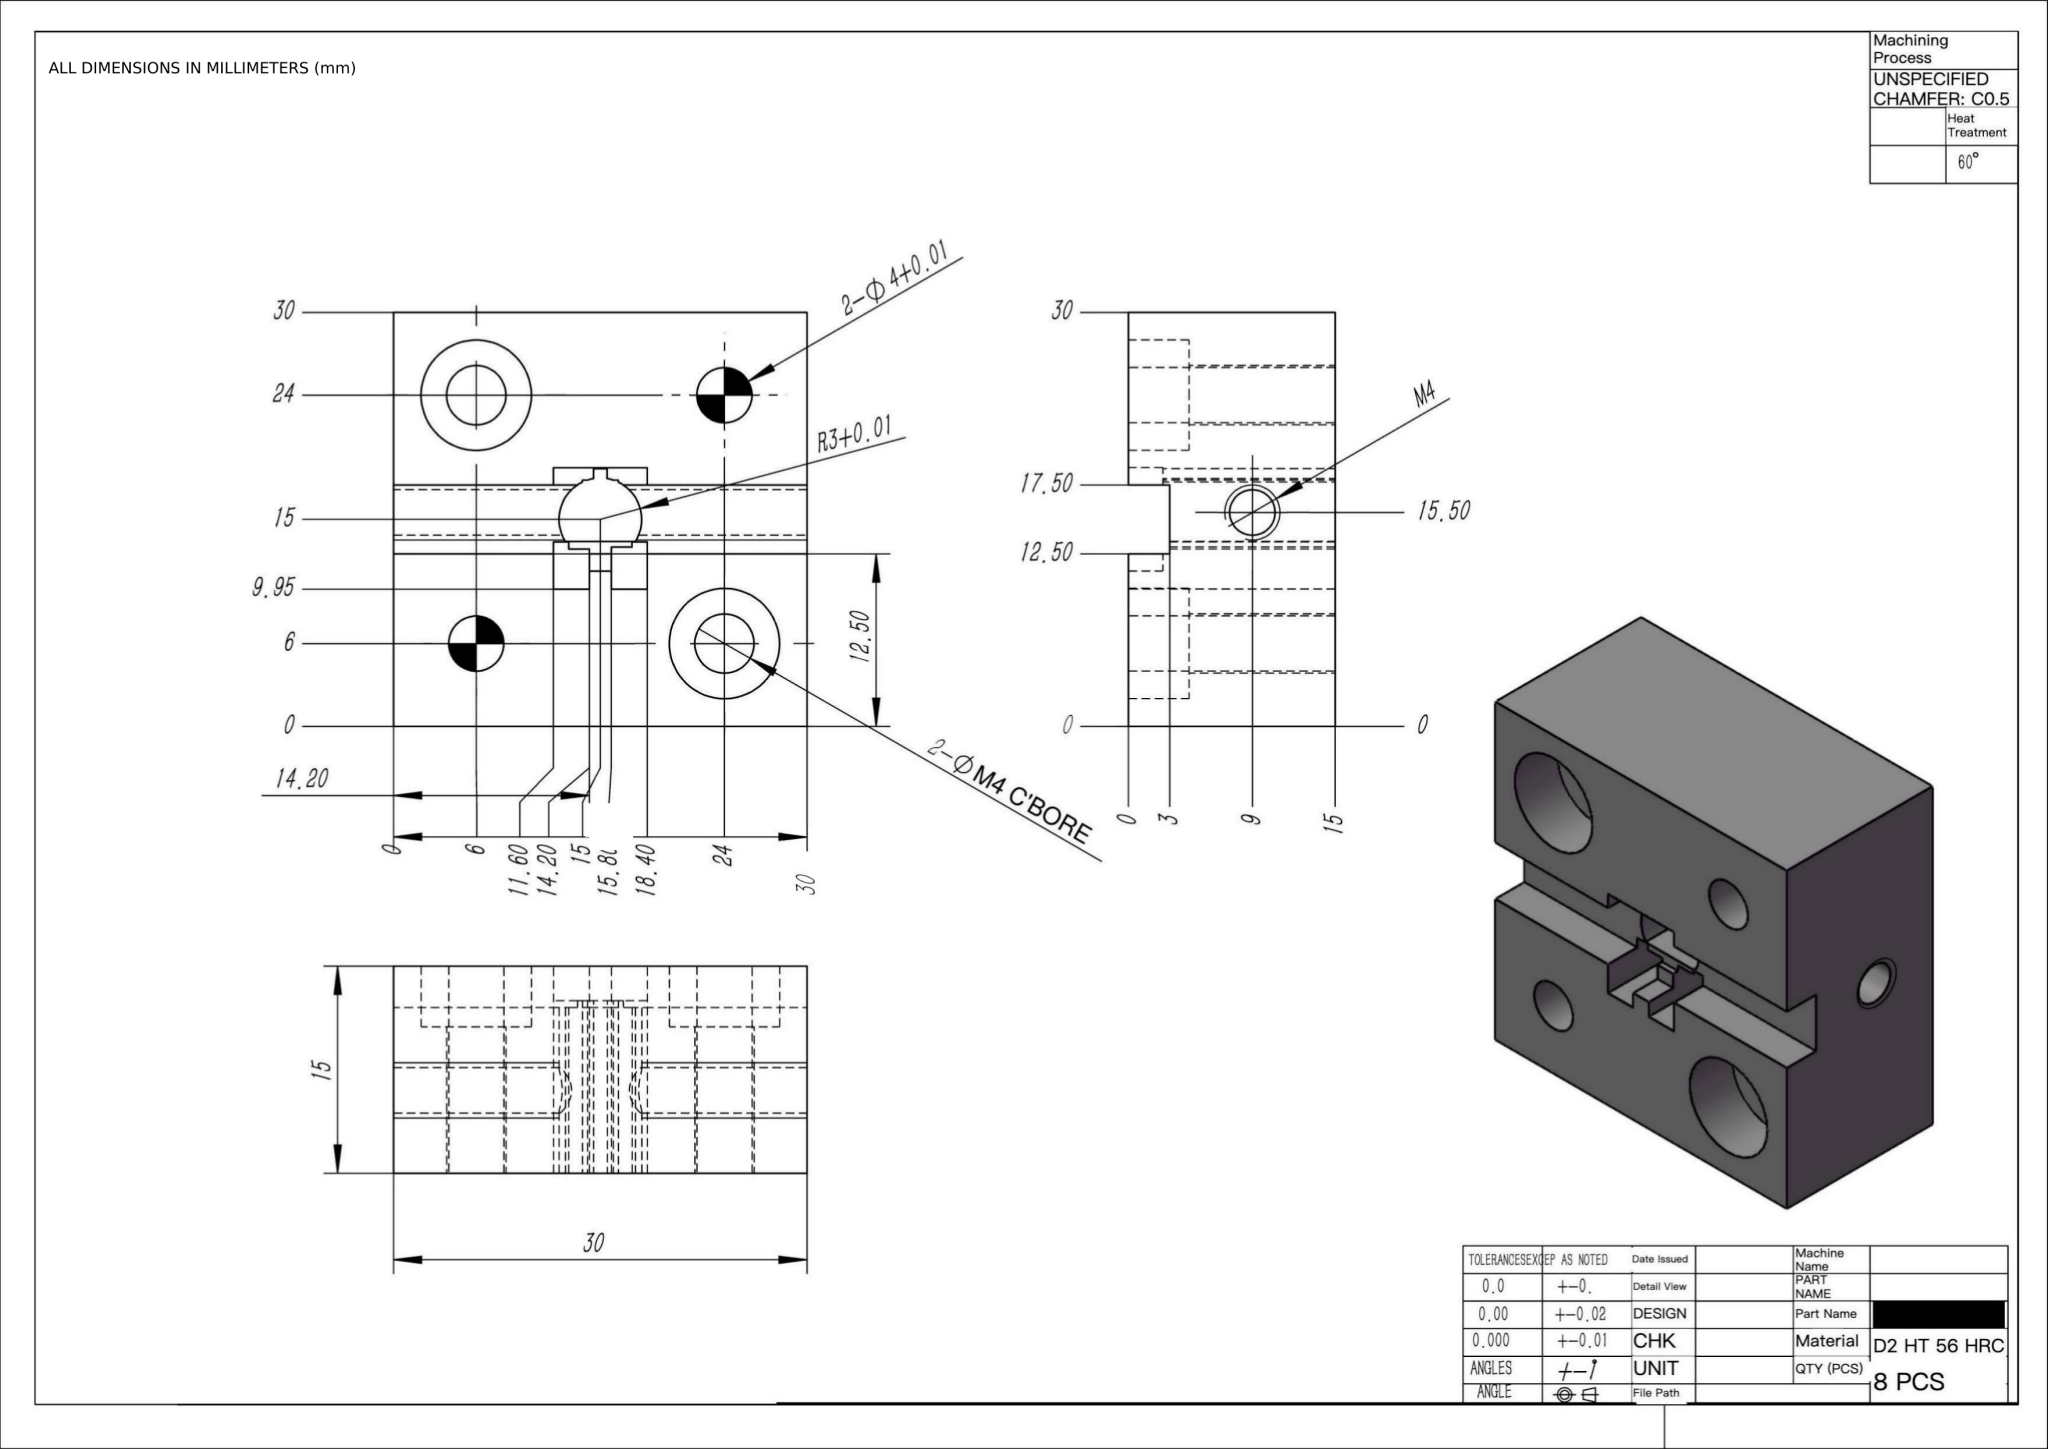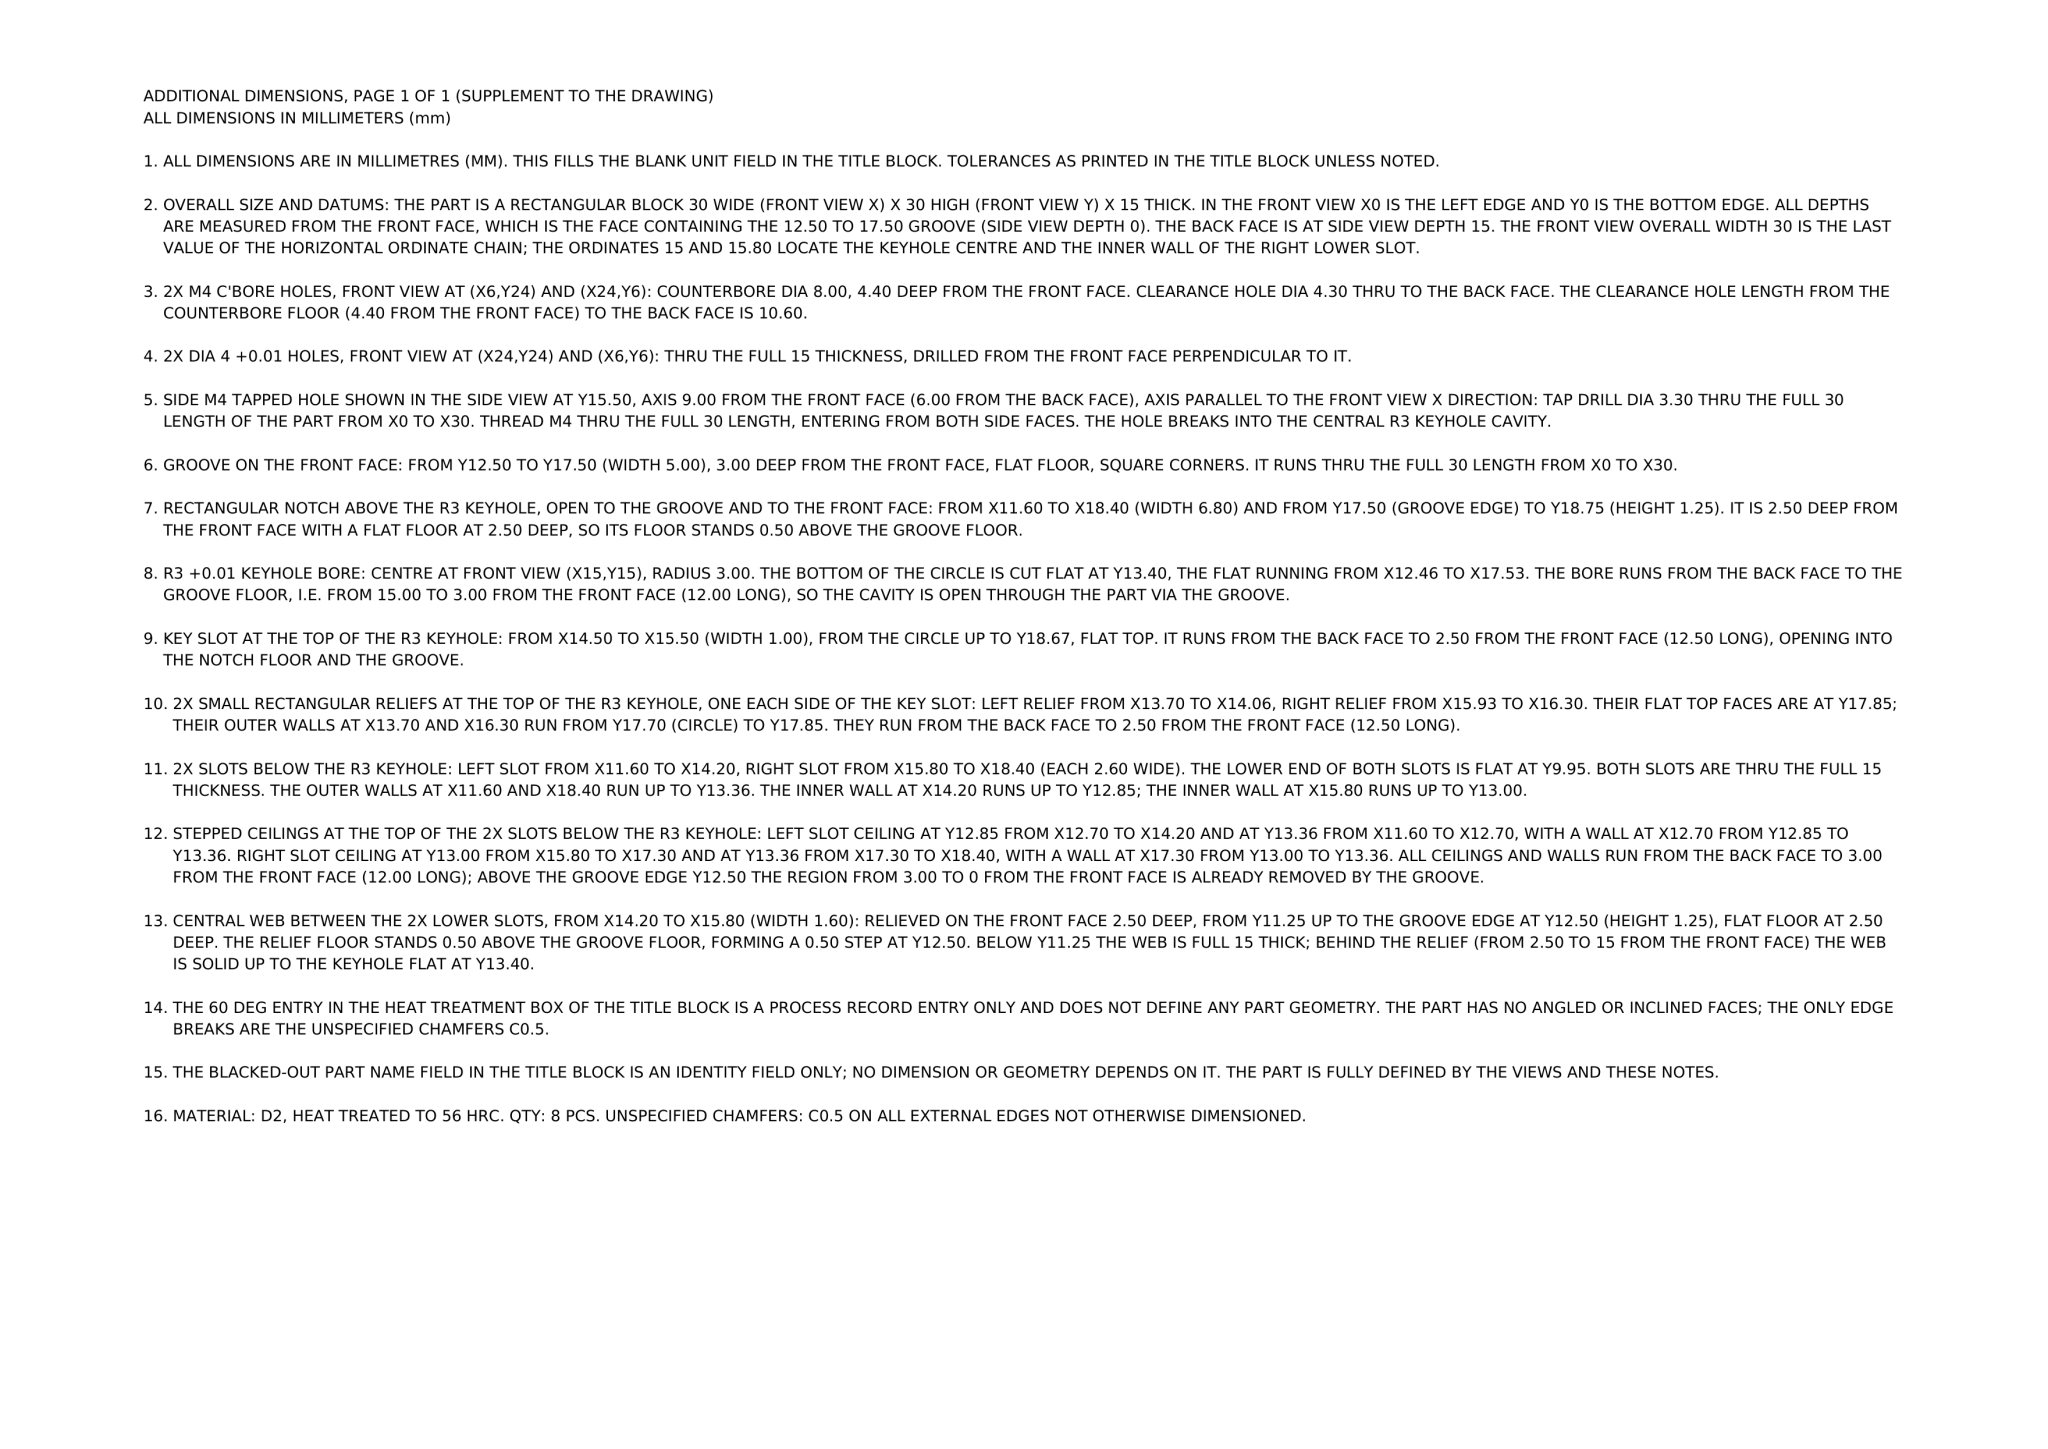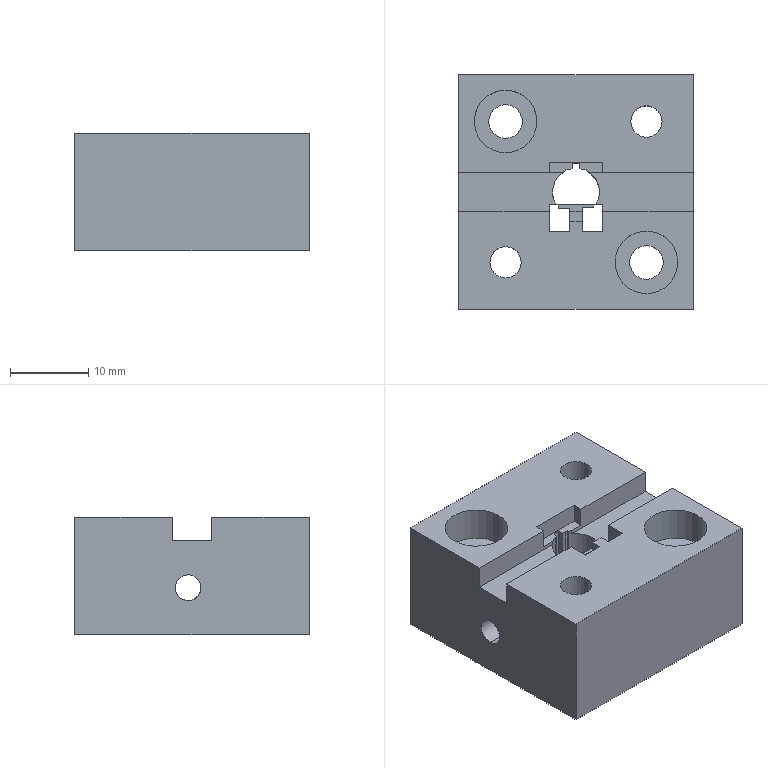Part | NX | mm | 1 solid | 62 faces | box 30 x 30 x 15 mm | volume 11163 mm3 | plane 41 | cylinder 21 | commonest cylinder face diameters 6 x5 3.3 x4 4 x4 8 x4 4.3 x4